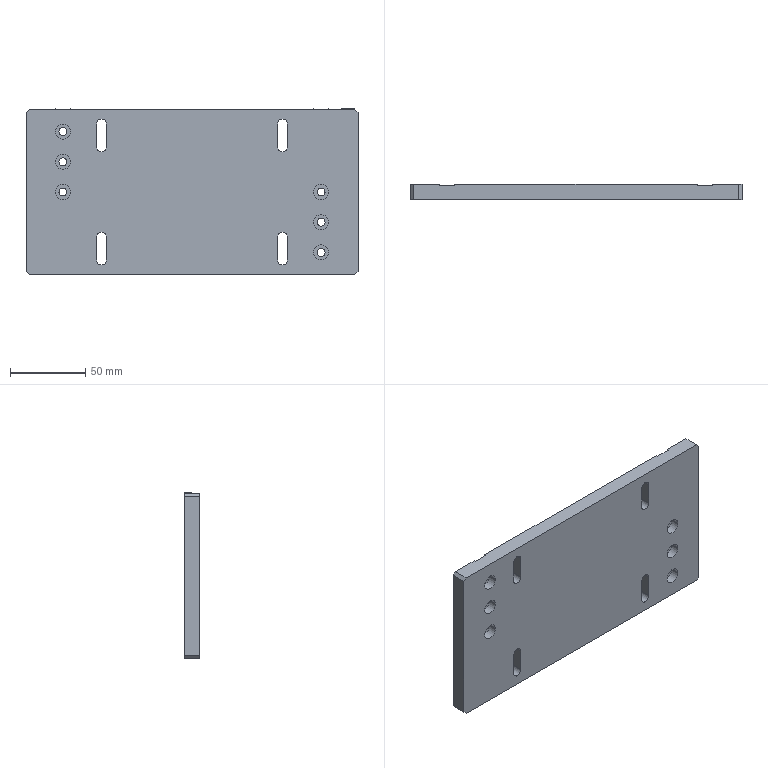Component | SolidWorks | AssemblyCylinderBracket54-1_BottomSupport-1 | 1 solid | 64 faces | box 220 x 10 x 110 mm | volume 231269 mm3 | cylinder 32 | plane 32 | commonest cylinder face diameters 10 x12 5.3 x12 6.6 x8
build123d program:
from build123d import *

# Parameters (mm, degrees)
SKETCH1_W                                          = 220
SKETCH1_H                                          = 110
BOSS_EXTRUDE1_DEPTH                                = 10
CHAMFER1_SIZE                                      = 2
CUT_EXTRUDE2_DEPTH                                 = 124.39
SKETCH6_W                                          = 10
SKETCH6_H                                          = 1
CUT_EXTRUDE3_DEPTH                                 = 156.885
HOLE_SIZE_ACCORDING_TO_HEX_SOCKET_HEAD_D           = 5.3
HOLE_SIZE_ACCORDING_TO_HEX_SOCKET_HEAD_DEPTH       = 10.1
HOLE_SIZE_ACCORDING_TO_HEX_SOCKET_HEAD_CBORE_D     = 10
HOLE_SIZE_ACCORDING_TO_HEX_SOCKET_HEAD_CBORE_DEPTH = 5.7
HOLE_SIZE_ACCORDING_TO_HEX_SOCKET_HEAD_TIP         = 1.592


with BuildPart() as part:
    # Sketch1 → Boss-Extrude1 (new body)
    with BuildSketch(Plane.XY):
        Rectangle(SKETCH1_W, SKETCH1_H)
    extrude(amount=BOSS_EXTRUDE1_DEPTH)

    # Chamfer1
    chamfer1_edges = [part.edges().sort_by_distance(p)[0] for p in [
        (110, -55, 5),
        (-110, -55, 5),
        (-110, 55, 5),
        (110, 55, 5),
    ]]
    chamfer(chamfer1_edges, length=CHAMFER1_SIZE)

    # Sketch5 → Cut-Extrude2 (cut, through all)
    with BuildSketch(Plane.XY.offset(10)):
        with BuildLine():
            Line((-56.7, 45), (-56.7, 30))
            ThreePointArc((-56.7, 30), (-60, 26.7), (-63.3, 30))
            Line((-63.3, 30), (-63.3, 45))
            ThreePointArc((-63.3, 45), (-60, 48.3), (-56.7, 45))
        make_face()
        with BuildLine():
            Line((-56.7, -45), (-56.7, -30))
            ThreePointArc((-56.7, -30), (-60, -26.7), (-63.3, -30))
            Line((-63.3, -30), (-63.3, -45))
            ThreePointArc((-63.3, -45), (-60, -48.3), (-56.7, -45))
        make_face()
        with BuildLine():
            Line((56.7, 45), (56.7, 30))
            ThreePointArc((56.7, 30), (60, 26.7), (63.3, 30))
            Line((63.3, 30), (63.3, 45))
            ThreePointArc((63.3, 45), (60, 48.3), (56.7, 45))
        make_face()
        with BuildLine():
            Line((56.7, -45), (56.7, -30))
            ThreePointArc((56.7, -30), (60, -26.7), (63.3, -30))
            Line((63.3, -30), (63.3, -45))
            ThreePointArc((63.3, -45), (60, -48.3), (56.7, -45))
        make_face()
    extrude(amount=-CUT_EXTRUDE2_DEPTH, mode=Mode.SUBTRACT)

    # Sketch6 → Cut-Extrude3 (cut, through all)
    with BuildSketch(Plane.XZ.offset(55)):
        with Locations((-85.5, 9.5)):
            Rectangle(SKETCH6_W, SKETCH6_H)
        with Locations((85.5, 9.5)):
            Rectangle(SKETCH6_W, SKETCH6_H)
    extrude(amount=-CUT_EXTRUDE3_DEPTH, mode=Mode.SUBTRACT)

    # Hole Size _According to_ Hex Socket Head
    with Locations(Plane(origin=(0, 0, 0), x_dir=(-1, 0, 0), z_dir=(0, 0, -1))):
        with Locations((85.5, -40), (85.5, -20), (85.5, 0), (-85.5, 20), (-85.5, 40), (-85.5, 0)):
            CounterBoreHole(HOLE_SIZE_ACCORDING_TO_HEX_SOCKET_HEAD_D / 2, HOLE_SIZE_ACCORDING_TO_HEX_SOCKET_HEAD_CBORE_D / 2, HOLE_SIZE_ACCORDING_TO_HEX_SOCKET_HEAD_CBORE_DEPTH, depth=HOLE_SIZE_ACCORDING_TO_HEX_SOCKET_HEAD_DEPTH)
            with Locations((0, 0, -(HOLE_SIZE_ACCORDING_TO_HEX_SOCKET_HEAD_DEPTH + HOLE_SIZE_ACCORDING_TO_HEX_SOCKET_HEAD_TIP / 2))):  # 118° drill point
                Cone(0, HOLE_SIZE_ACCORDING_TO_HEX_SOCKET_HEAD_D / 2, HOLE_SIZE_ACCORDING_TO_HEX_SOCKET_HEAD_TIP, mode=Mode.SUBTRACT)


solid = part.part

# Placed as in the assembly
solid = solid.moved(Location((54.585, -127.305, 51.359), (-90, 0, 0)))